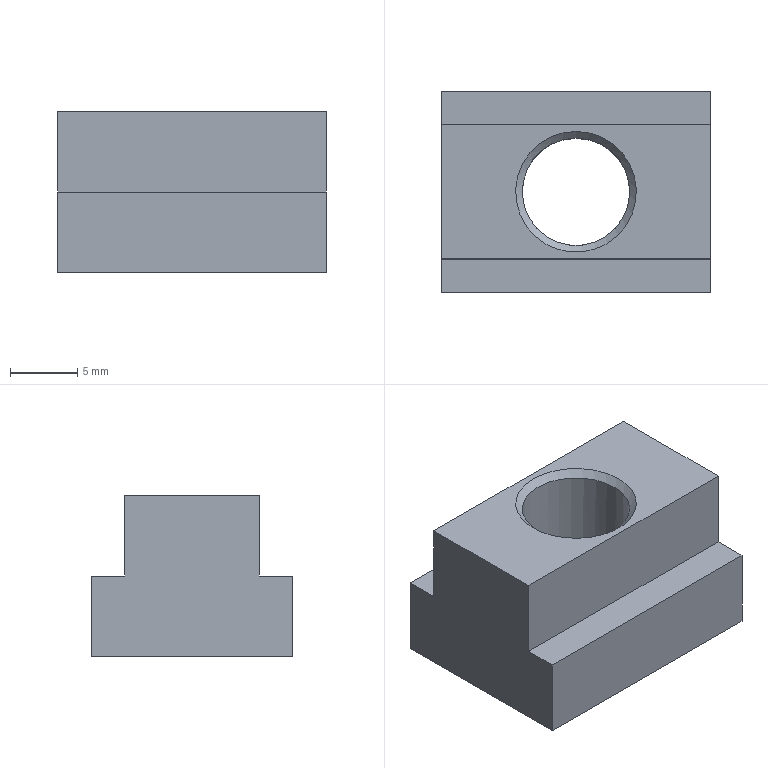Component | NX | FIXED_BLOCK | 1 solid | 13 faces | box 20 x 15 x 12 mm | volume 2390 mm3 | plane 10 | cone 2 | cylinder 1 | commonest cylinder face diameters 8 x1
STEP:
#1=CARTESIAN_POINT('',(0.,0.,0.));
#2=DIRECTION('',(0.,0.,1.));
#3=DIRECTION('',(1.,0.,0.));
#4=AXIS2_PLACEMENT_3D('',#1,#2,#3);
#5=CARTESIAN_POINT('',(-305.,-127.5,4.5));
#6=VERTEX_POINT('',#5);
#7=CARTESIAN_POINT('',(-305.,-127.5,-1.5));
#8=VERTEX_POINT('',#7);
#9=CARTESIAN_POINT('',(-305.,-127.5,4.5));
#10=DIRECTION('',(0.,0.,-1.));
#11=VECTOR('',#10,1.);
#12=LINE('',#9,#11);
#13=CARTESIAN_POINT('',(-285.,-127.5,4.5));
#14=DIRECTION('',(0.,1.,0.));
#15=DIRECTION('',(0.,0.,1.));
#16=AXIS2_PLACEMENT_3D('',#13,#14,#15);
#17=PLANE('',#16);
#18=CARTESIAN_POINT('',(0.,-20.));
#19=DIRECTION('',(-1.,0.));
#20=VECTOR('',#19,1.);
#21=LINE('',#18,#20);
#22=(GEOMETRIC_REPRESENTATION_CONTEXT(2)PARAMETRIC_REPRESENTATION_CONTEXT()REPRESENTATION_CONTEXT('',''));
#23=DEFINITIONAL_REPRESENTATION('',(#21),#22);
#24=PCURVE('',#17,#23);
#25=CARTESIAN_POINT('',(-305.,-120.,10.5));
#26=DIRECTION('',(1.,0.,0.));
#27=DIRECTION('',(0.,0.,-1.));
#28=AXIS2_PLACEMENT_3D('',#25,#26,#27);
#29=PLANE('',#28);
#30=CARTESIAN_POINT('',(6.,-7.5));
#31=DIRECTION('',(1.,0.));
#32=VECTOR('',#31,1.);
#33=LINE('',#30,#32);
#34=(GEOMETRIC_REPRESENTATION_CONTEXT(2)PARAMETRIC_REPRESENTATION_CONTEXT()REPRESENTATION_CONTEXT('',''));
#35=DEFINITIONAL_REPRESENTATION('',(#33),#34);
#36=PCURVE('',#29,#35);
#37=SURFACE_CURVE('',#12,(#24,#36),.PCURVE_S1.);
#38=EDGE_CURVE('',#6,#8,#37,.T.);
#39=ORIENTED_EDGE('',*,*,#38,.T.);
#40=CARTESIAN_POINT('',(-285.,-127.5,-1.5));
#41=VERTEX_POINT('',#40);
#42=CARTESIAN_POINT('',(-285.,-127.5,-1.5));
#43=DIRECTION('',(-1.,0.,0.));
#44=VECTOR('',#43,1.);
#45=LINE('',#42,#44);
#46=CARTESIAN_POINT('',(-6.,0.));
#47=DIRECTION('',(0.,-1.));
#48=VECTOR('',#47,1.);
#49=LINE('',#46,#48);
#50=(GEOMETRIC_REPRESENTATION_CONTEXT(2)PARAMETRIC_REPRESENTATION_CONTEXT()REPRESENTATION_CONTEXT('',''));
#51=DEFINITIONAL_REPRESENTATION('',(#49),#50);
#52=PCURVE('',#17,#51);
#53=CARTESIAN_POINT('',(-285.,-120.,-1.5));
#54=DIRECTION('',(0.,0.,1.));
#55=DIRECTION('',(1.,0.,0.));
#56=AXIS2_PLACEMENT_3D('',#53,#54,#55);
#57=PLANE('',#56);
#58=CARTESIAN_POINT('',(0.,-7.5));
#59=DIRECTION('',(-1.,0.));
#60=VECTOR('',#59,1.);
#61=LINE('',#58,#60);
#62=(GEOMETRIC_REPRESENTATION_CONTEXT(2)PARAMETRIC_REPRESENTATION_CONTEXT()REPRESENTATION_CONTEXT('',''));
#63=DEFINITIONAL_REPRESENTATION('',(#61),#62);
#64=PCURVE('',#57,#63);
#65=SURFACE_CURVE('',#45,(#52,#64),.PCURVE_S1.);
#66=EDGE_CURVE('',#41,#8,#65,.T.);
#67=ORIENTED_EDGE('',*,*,#66,.F.);
#68=CARTESIAN_POINT('',(-285.,-127.5,4.5));
#69=VERTEX_POINT('',#68);
#70=CARTESIAN_POINT('',(-285.,-127.5,4.5));
#71=DIRECTION('',(0.,0.,-1.));
#72=VECTOR('',#71,1.);
#73=LINE('',#70,#72);
#74=CARTESIAN_POINT('',(0.,0.));
#75=DIRECTION('',(-1.,0.));
#76=VECTOR('',#75,1.);
#77=LINE('',#74,#76);
#78=(GEOMETRIC_REPRESENTATION_CONTEXT(2)PARAMETRIC_REPRESENTATION_CONTEXT()REPRESENTATION_CONTEXT('',''));
#79=DEFINITIONAL_REPRESENTATION('',(#77),#78);
#80=PCURVE('',#17,#79);
#81=CARTESIAN_POINT('',(-285.,-120.,10.5));
#82=DIRECTION('',(1.,0.,0.));
#83=DIRECTION('',(0.,0.,-1.));
#84=AXIS2_PLACEMENT_3D('',#81,#82,#83);
#85=PLANE('',#84);
#86=CARTESIAN_POINT('',(6.,-7.5));
#87=DIRECTION('',(1.,0.));
#88=VECTOR('',#87,1.);
#89=LINE('',#86,#88);
#90=(GEOMETRIC_REPRESENTATION_CONTEXT(2)PARAMETRIC_REPRESENTATION_CONTEXT()REPRESENTATION_CONTEXT('',''));
#91=DEFINITIONAL_REPRESENTATION('',(#89),#90);
#92=PCURVE('',#85,#91);
#93=SURFACE_CURVE('',#73,(#80,#92),.PCURVE_S1.);
#94=EDGE_CURVE('',#69,#41,#93,.T.);
#95=ORIENTED_EDGE('',*,*,#94,.F.);
#96=CARTESIAN_POINT('',(-285.,-127.5,4.5));
#97=DIRECTION('',(-1.,0.,0.));
#98=VECTOR('',#97,1.);
#99=LINE('',#96,#98);
#100=CARTESIAN_POINT('',(0.,0.));
#101=DIRECTION('',(0.,-1.));
#102=VECTOR('',#101,1.);
#103=LINE('',#100,#102);
#104=(GEOMETRIC_REPRESENTATION_CONTEXT(2)PARAMETRIC_REPRESENTATION_CONTEXT()REPRESENTATION_CONTEXT('',''));
#105=DEFINITIONAL_REPRESENTATION('',(#103),#104);
#106=PCURVE('',#17,#105);
#107=CARTESIAN_POINT('',(-285.,-125.,4.5));
#108=DIRECTION('',(0.,0.,-1.));
#109=DIRECTION('',(0.,1.,0.));
#110=AXIS2_PLACEMENT_3D('',#107,#108,#109);
#111=PLANE('',#110);
#112=CARTESIAN_POINT('',(-2.5,0.));
#113=DIRECTION('',(0.,-1.));
#114=VECTOR('',#113,1.);
#115=LINE('',#112,#114);
#116=(GEOMETRIC_REPRESENTATION_CONTEXT(2)PARAMETRIC_REPRESENTATION_CONTEXT()REPRESENTATION_CONTEXT('',''));
#117=DEFINITIONAL_REPRESENTATION('',(#115),#116);
#118=PCURVE('',#111,#117);
#119=SURFACE_CURVE('',#99,(#106,#118),.PCURVE_S1.);
#120=EDGE_CURVE('',#69,#6,#119,.T.);
#121=ORIENTED_EDGE('',*,*,#120,.T.);
#122=EDGE_LOOP('',(#39,#67,#95,#121));
#123=FACE_BOUND('',#122,.T.);
#124=ADVANCED_FACE('',(#123),#17,.F.);
#125=CARTESIAN_POINT('',(-290.5,-120.,-1.5));
#126=VERTEX_POINT('',#125);
#127=CARTESIAN_POINT('',(-295.,-115.5,-1.5));
#128=VERTEX_POINT('',#127);
#129=CARTESIAN_POINT('',(-295.,-120.,-1.5));
#130=DIRECTION('',(0.,0.,1.));
#131=DIRECTION('',(1.,0.,0.));
#132=AXIS2_PLACEMENT_3D('',#129,#130,#131);
#133=CIRCLE('',#132,4.5);
#134=CARTESIAN_POINT('',(-10.,0.));
#135=DIRECTION('',(1.,0.));
#136=AXIS2_PLACEMENT_2D('',#134,#135);
#137=CIRCLE('',#136,4.5);
#138=(GEOMETRIC_REPRESENTATION_CONTEXT(2)PARAMETRIC_REPRESENTATION_CONTEXT()REPRESENTATION_CONTEXT('',''));
#139=DEFINITIONAL_REPRESENTATION('',(#137),#138);
#140=PCURVE('',#57,#139);
#141=CARTESIAN_POINT('',(-295.,-120.,-1.5));
#142=DIRECTION('',(0.,0.,-1.));
#143=DIRECTION('',(0.,1.,0.));
#144=AXIS2_PLACEMENT_3D('',#141,#142,#143);
#145=CONICAL_SURFACE('',#144,4.5,0.7854);
#146=CARTESIAN_POINT('',(1.571,0.));
#147=DIRECTION('',(-1.,0.));
#148=VECTOR('',#147,1.);
#149=LINE('',#146,#148);
#150=(GEOMETRIC_REPRESENTATION_CONTEXT(2)PARAMETRIC_REPRESENTATION_CONTEXT()REPRESENTATION_CONTEXT('',''));
#151=DEFINITIONAL_REPRESENTATION('',(#149),#150);
#152=PCURVE('',#145,#151);
#153=SURFACE_CURVE('',#133,(#140,#152),.PCURVE_S1.);
#154=EDGE_CURVE('',#126,#128,#153,.T.);
#155=ORIENTED_EDGE('',*,*,#154,.T.);
#156=CARTESIAN_POINT('',(-295.,-120.,-1.5));
#157=DIRECTION('',(0.,0.,1.));
#158=DIRECTION('',(1.,0.,0.));
#159=AXIS2_PLACEMENT_3D('',#156,#157,#158);
#160=CIRCLE('',#159,4.5);
#161=CARTESIAN_POINT('',(-10.,0.));
#162=DIRECTION('',(1.,0.));
#163=AXIS2_PLACEMENT_2D('',#161,#162);
#164=CIRCLE('',#163,4.5);
#165=(GEOMETRIC_REPRESENTATION_CONTEXT(2)PARAMETRIC_REPRESENTATION_CONTEXT()REPRESENTATION_CONTEXT('',''));
#166=DEFINITIONAL_REPRESENTATION('',(#164),#165);
#167=PCURVE('',#57,#166);
#168=CARTESIAN_POINT('',(7.854,0.));
#169=DIRECTION('',(-1.,0.));
#170=VECTOR('',#169,1.);
#171=LINE('',#168,#170);
#172=(GEOMETRIC_REPRESENTATION_CONTEXT(2)PARAMETRIC_REPRESENTATION_CONTEXT()REPRESENTATION_CONTEXT('',''));
#173=DEFINITIONAL_REPRESENTATION('',(#171),#172);
#174=PCURVE('',#145,#173);
#175=SURFACE_CURVE('',#160,(#167,#174),.PCURVE_S1.);
#176=EDGE_CURVE('',#128,#126,#175,.T.);
#177=ORIENTED_EDGE('',*,*,#176,.T.);
#178=EDGE_LOOP('',(#155,#177));
#179=FACE_BOUND('',#178,.T.);
#180=CARTESIAN_POINT('',(-305.,-112.5,-1.5));
#181=VERTEX_POINT('',#180);
#182=CARTESIAN_POINT('',(-305.,-120.,-1.5));
#183=DIRECTION('',(0.,1.,0.));
#184=VECTOR('',#183,1.);
#185=LINE('',#182,#184);
#186=CARTESIAN_POINT('',(-20.,0.));
#187=DIRECTION('',(0.,1.));
#188=VECTOR('',#187,1.);
#189=LINE('',#186,#188);
#190=(GEOMETRIC_REPRESENTATION_CONTEXT(2)PARAMETRIC_REPRESENTATION_CONTEXT()REPRESENTATION_CONTEXT('',''));
#191=DEFINITIONAL_REPRESENTATION('',(#189),#190);
#192=PCURVE('',#57,#191);
#193=CARTESIAN_POINT('',(12.,0.));
#194=DIRECTION('',(0.,1.));
#195=VECTOR('',#194,1.);
#196=LINE('',#193,#195);
#197=(GEOMETRIC_REPRESENTATION_CONTEXT(2)PARAMETRIC_REPRESENTATION_CONTEXT()REPRESENTATION_CONTEXT('',''));
#198=DEFINITIONAL_REPRESENTATION('',(#196),#197);
#199=PCURVE('',#29,#198);
#200=SURFACE_CURVE('',#185,(#192,#199),.PCURVE_S1.);
#201=EDGE_CURVE('',#8,#181,#200,.T.);
#202=ORIENTED_EDGE('',*,*,#201,.T.);
#203=CARTESIAN_POINT('',(-285.,-112.5,-1.5));
#204=VERTEX_POINT('',#203);
#205=CARTESIAN_POINT('',(-285.,-112.5,-1.5));
#206=DIRECTION('',(-1.,0.,0.));
#207=VECTOR('',#206,1.);
#208=LINE('',#205,#207);
#209=CARTESIAN_POINT('',(0.,7.5));
#210=DIRECTION('',(-1.,0.));
#211=VECTOR('',#210,1.);
#212=LINE('',#209,#211);
#213=(GEOMETRIC_REPRESENTATION_CONTEXT(2)PARAMETRIC_REPRESENTATION_CONTEXT()REPRESENTATION_CONTEXT('',''));
#214=DEFINITIONAL_REPRESENTATION('',(#212),#213);
#215=PCURVE('',#57,#214);
#216=CARTESIAN_POINT('',(-285.,-112.5,-1.5));
#217=DIRECTION('',(0.,-1.,0.));
#218=DIRECTION('',(0.,0.,-1.));
#219=AXIS2_PLACEMENT_3D('',#216,#217,#218);
#220=PLANE('',#219);
#221=CARTESIAN_POINT('',(0.,0.));
#222=DIRECTION('',(0.,-1.));
#223=VECTOR('',#222,1.);
#224=LINE('',#221,#223);
#225=(GEOMETRIC_REPRESENTATION_CONTEXT(2)PARAMETRIC_REPRESENTATION_CONTEXT()REPRESENTATION_CONTEXT('',''));
#226=DEFINITIONAL_REPRESENTATION('',(#224),#225);
#227=PCURVE('',#220,#226);
#228=SURFACE_CURVE('',#208,(#215,#227),.PCURVE_S1.);
#229=EDGE_CURVE('',#204,#181,#228,.T.);
#230=ORIENTED_EDGE('',*,*,#229,.F.);
#231=CARTESIAN_POINT('',(-285.,-127.5,-1.5));
#232=DIRECTION('',(0.,1.,0.));
#233=VECTOR('',#232,1.);
#234=LINE('',#231,#233);
#235=CARTESIAN_POINT('',(0.,-7.5));
#236=DIRECTION('',(0.,1.));
#237=VECTOR('',#236,1.);
#238=LINE('',#235,#237);
#239=(GEOMETRIC_REPRESENTATION_CONTEXT(2)PARAMETRIC_REPRESENTATION_CONTEXT()REPRESENTATION_CONTEXT('',''));
#240=DEFINITIONAL_REPRESENTATION('',(#238),#239);
#241=PCURVE('',#57,#240);
#242=CARTESIAN_POINT('',(12.,-7.5));
#243=DIRECTION('',(0.,1.));
#244=VECTOR('',#243,1.);
#245=LINE('',#242,#244);
#246=(GEOMETRIC_REPRESENTATION_CONTEXT(2)PARAMETRIC_REPRESENTATION_CONTEXT()REPRESENTATION_CONTEXT('',''));
#247=DEFINITIONAL_REPRESENTATION('',(#245),#246);
#248=PCURVE('',#85,#247);
#249=SURFACE_CURVE('',#234,(#241,#248),.PCURVE_S1.);
#250=EDGE_CURVE('',#41,#204,#249,.T.);
#251=ORIENTED_EDGE('',*,*,#250,.F.);
#252=ORIENTED_EDGE('',*,*,#66,.T.);
#253=EDGE_LOOP('',(#202,#230,#251,#252));
#254=FACE_BOUND('',#253,.T.);
#255=ADVANCED_FACE('',(#179,#254),#57,.F.);
#256=CARTESIAN_POINT('',(-305.,-112.5,4.5));
#257=VERTEX_POINT('',#256);
#258=CARTESIAN_POINT('',(-305.,-112.5,-1.5));
#259=DIRECTION('',(0.,0.,1.));
#260=VECTOR('',#259,1.);
#261=LINE('',#258,#260);
#262=CARTESIAN_POINT('',(0.,-20.));
#263=DIRECTION('',(-1.,0.));
#264=VECTOR('',#263,1.);
#265=LINE('',#262,#264);
#266=(GEOMETRIC_REPRESENTATION_CONTEXT(2)PARAMETRIC_REPRESENTATION_CONTEXT()REPRESENTATION_CONTEXT('',''));
#267=DEFINITIONAL_REPRESENTATION('',(#265),#266);
#268=PCURVE('',#220,#267);
#269=CARTESIAN_POINT('',(12.,7.5));
#270=DIRECTION('',(-1.,0.));
#271=VECTOR('',#270,1.);
#272=LINE('',#269,#271);
#273=(GEOMETRIC_REPRESENTATION_CONTEXT(2)PARAMETRIC_REPRESENTATION_CONTEXT()REPRESENTATION_CONTEXT('',''));
#274=DEFINITIONAL_REPRESENTATION('',(#272),#273);
#275=PCURVE('',#29,#274);
#276=SURFACE_CURVE('',#261,(#268,#275),.PCURVE_S1.);
#277=EDGE_CURVE('',#181,#257,#276,.T.);
#278=ORIENTED_EDGE('',*,*,#277,.T.);
#279=CARTESIAN_POINT('',(-285.,-112.5,4.5));
#280=VERTEX_POINT('',#279);
#281=CARTESIAN_POINT('',(-285.,-112.5,4.5));
#282=DIRECTION('',(-1.,0.,0.));
#283=VECTOR('',#282,1.);
#284=LINE('',#281,#283);
#285=CARTESIAN_POINT('',(-6.,0.));
#286=DIRECTION('',(0.,-1.));
#287=VECTOR('',#286,1.);
#288=LINE('',#285,#287);
#289=(GEOMETRIC_REPRESENTATION_CONTEXT(2)PARAMETRIC_REPRESENTATION_CONTEXT()REPRESENTATION_CONTEXT('',''));
#290=DEFINITIONAL_REPRESENTATION('',(#288),#289);
#291=PCURVE('',#220,#290);
#292=CARTESIAN_POINT('',(-285.,-112.5,4.5));
#293=DIRECTION('',(0.,-0.,-1.));
#294=DIRECTION('',(0.,1.,-0.));
#295=AXIS2_PLACEMENT_3D('',#292,#293,#294);
#296=PLANE('',#295);
#297=CARTESIAN_POINT('',(0.,0.));
#298=DIRECTION('',(0.,-1.));
#299=VECTOR('',#298,1.);
#300=LINE('',#297,#299);
#301=(GEOMETRIC_REPRESENTATION_CONTEXT(2)PARAMETRIC_REPRESENTATION_CONTEXT()REPRESENTATION_CONTEXT('',''));
#302=DEFINITIONAL_REPRESENTATION('',(#300),#301);
#303=PCURVE('',#296,#302);
#304=SURFACE_CURVE('',#284,(#291,#303),.PCURVE_S1.);
#305=EDGE_CURVE('',#280,#257,#304,.T.);
#306=ORIENTED_EDGE('',*,*,#305,.F.);
#307=CARTESIAN_POINT('',(-285.,-112.5,-1.5));
#308=DIRECTION('',(0.,0.,1.));
#309=VECTOR('',#308,1.);
#310=LINE('',#307,#309);
#311=CARTESIAN_POINT('',(0.,0.));
#312=DIRECTION('',(-1.,0.));
#313=VECTOR('',#312,1.);
#314=LINE('',#311,#313);
#315=(GEOMETRIC_REPRESENTATION_CONTEXT(2)PARAMETRIC_REPRESENTATION_CONTEXT()REPRESENTATION_CONTEXT('',''));
#316=DEFINITIONAL_REPRESENTATION('',(#314),#315);
#317=PCURVE('',#220,#316);
#318=CARTESIAN_POINT('',(12.,7.5));
#319=DIRECTION('',(-1.,0.));
#320=VECTOR('',#319,1.);
#321=LINE('',#318,#320);
#322=(GEOMETRIC_REPRESENTATION_CONTEXT(2)PARAMETRIC_REPRESENTATION_CONTEXT()REPRESENTATION_CONTEXT('',''));
#323=DEFINITIONAL_REPRESENTATION('',(#321),#322);
#324=PCURVE('',#85,#323);
#325=SURFACE_CURVE('',#310,(#317,#324),.PCURVE_S1.);
#326=EDGE_CURVE('',#204,#280,#325,.T.);
#327=ORIENTED_EDGE('',*,*,#326,.F.);
#328=ORIENTED_EDGE('',*,*,#229,.T.);
#329=EDGE_LOOP('',(#278,#306,#327,#328));
#330=FACE_BOUND('',#329,.T.);
#331=ADVANCED_FACE('',(#330),#220,.F.);
#332=CARTESIAN_POINT('',(-305.,-115.,4.5));
#333=VERTEX_POINT('',#332);
#334=CARTESIAN_POINT('',(-305.,-112.5,4.5));
#335=DIRECTION('',(0.,-1.,0.));
#336=VECTOR('',#335,1.);
#337=LINE('',#334,#336);
#338=CARTESIAN_POINT('',(0.,-20.));
#339=DIRECTION('',(-1.,0.));
#340=VECTOR('',#339,1.);
#341=LINE('',#338,#340);
#342=(GEOMETRIC_REPRESENTATION_CONTEXT(2)PARAMETRIC_REPRESENTATION_CONTEXT()REPRESENTATION_CONTEXT('',''));
#343=DEFINITIONAL_REPRESENTATION('',(#341),#342);
#344=PCURVE('',#296,#343);
#345=CARTESIAN_POINT('',(6.,7.5));
#346=DIRECTION('',(-0.,-1.));
#347=VECTOR('',#346,1.);
#348=LINE('',#345,#347);
#349=(GEOMETRIC_REPRESENTATION_CONTEXT(2)PARAMETRIC_REPRESENTATION_CONTEXT()REPRESENTATION_CONTEXT('',''));
#350=DEFINITIONAL_REPRESENTATION('',(#348),#349);
#351=PCURVE('',#29,#350);
#352=SURFACE_CURVE('',#337,(#344,#351),.PCURVE_S1.);
#353=EDGE_CURVE('',#257,#333,#352,.T.);
#354=ORIENTED_EDGE('',*,*,#353,.T.);
#355=CARTESIAN_POINT('',(-285.,-115.,4.5));
#356=VERTEX_POINT('',#355);
#357=CARTESIAN_POINT('',(-285.,-115.,4.5));
#358=DIRECTION('',(-1.,0.,0.));
#359=VECTOR('',#358,1.);
#360=LINE('',#357,#359);
#361=CARTESIAN_POINT('',(-2.5,0.));
#362=DIRECTION('',(0.,-1.));
#363=VECTOR('',#362,1.);
#364=LINE('',#361,#363);
#365=(GEOMETRIC_REPRESENTATION_CONTEXT(2)PARAMETRIC_REPRESENTATION_CONTEXT()REPRESENTATION_CONTEXT('',''));
#366=DEFINITIONAL_REPRESENTATION('',(#364),#365);
#367=PCURVE('',#296,#366);
#368=CARTESIAN_POINT('',(-285.,-115.,4.5));
#369=DIRECTION('',(0.,-1.,0.));
#370=DIRECTION('',(0.,0.,-1.));
#371=AXIS2_PLACEMENT_3D('',#368,#369,#370);
#372=PLANE('',#371);
#373=CARTESIAN_POINT('',(0.,0.));
#374=DIRECTION('',(0.,-1.));
#375=VECTOR('',#374,1.);
#376=LINE('',#373,#375);
#377=(GEOMETRIC_REPRESENTATION_CONTEXT(2)PARAMETRIC_REPRESENTATION_CONTEXT()REPRESENTATION_CONTEXT('',''));
#378=DEFINITIONAL_REPRESENTATION('',(#376),#377);
#379=PCURVE('',#372,#378);
#380=SURFACE_CURVE('',#360,(#367,#379),.PCURVE_S1.);
#381=EDGE_CURVE('',#356,#333,#380,.T.);
#382=ORIENTED_EDGE('',*,*,#381,.F.);
#383=CARTESIAN_POINT('',(-285.,-112.5,4.5));
#384=DIRECTION('',(0.,-1.,0.));
#385=VECTOR('',#384,1.);
#386=LINE('',#383,#385);
#387=CARTESIAN_POINT('',(0.,0.));
#388=DIRECTION('',(-1.,0.));
#389=VECTOR('',#388,1.);
#390=LINE('',#387,#389);
#391=(GEOMETRIC_REPRESENTATION_CONTEXT(2)PARAMETRIC_REPRESENTATION_CONTEXT()REPRESENTATION_CONTEXT('',''));
#392=DEFINITIONAL_REPRESENTATION('',(#390),#391);
#393=PCURVE('',#296,#392);
#394=CARTESIAN_POINT('',(6.,7.5));
#395=DIRECTION('',(-0.,-1.));
#396=VECTOR('',#395,1.);
#397=LINE('',#394,#396);
#398=(GEOMETRIC_REPRESENTATION_CONTEXT(2)PARAMETRIC_REPRESENTATION_CONTEXT()REPRESENTATION_CONTEXT('',''));
#399=DEFINITIONAL_REPRESENTATION('',(#397),#398);
#400=PCURVE('',#85,#399);
#401=SURFACE_CURVE('',#386,(#393,#400),.PCURVE_S1.);
#402=EDGE_CURVE('',#280,#356,#401,.T.);
#403=ORIENTED_EDGE('',*,*,#402,.F.);
#404=ORIENTED_EDGE('',*,*,#305,.T.);
#405=EDGE_LOOP('',(#354,#382,#403,#404));
#406=FACE_BOUND('',#405,.T.);
#407=ADVANCED_FACE('',(#406),#296,.F.);
#408=CARTESIAN_POINT('',(-305.,-115.,10.5));
#409=VERTEX_POINT('',#408);
#410=CARTESIAN_POINT('',(-305.,-115.,4.5));
#411=DIRECTION('',(0.,0.,1.));
#412=VECTOR('',#411,1.);
#413=LINE('',#410,#412);
#414=CARTESIAN_POINT('',(0.,-20.));
#415=DIRECTION('',(-1.,0.));
#416=VECTOR('',#415,1.);
#417=LINE('',#414,#416);
#418=(GEOMETRIC_REPRESENTATION_CONTEXT(2)PARAMETRIC_REPRESENTATION_CONTEXT()REPRESENTATION_CONTEXT('',''));
#419=DEFINITIONAL_REPRESENTATION('',(#417),#418);
#420=PCURVE('',#372,#419);
#421=CARTESIAN_POINT('',(6.,5.));
#422=DIRECTION('',(-1.,0.));
#423=VECTOR('',#422,1.);
#424=LINE('',#421,#423);
#425=(GEOMETRIC_REPRESENTATION_CONTEXT(2)PARAMETRIC_REPRESENTATION_CONTEXT()REPRESENTATION_CONTEXT('',''));
#426=DEFINITIONAL_REPRESENTATION('',(#424),#425);
#427=PCURVE('',#29,#426);
#428=SURFACE_CURVE('',#413,(#420,#427),.PCURVE_S1.);
#429=EDGE_CURVE('',#333,#409,#428,.T.);
#430=ORIENTED_EDGE('',*,*,#429,.T.);
#431=CARTESIAN_POINT('',(-285.,-115.,10.5));
#432=VERTEX_POINT('',#431);
#433=CARTESIAN_POINT('',(-285.,-115.,10.5));
#434=DIRECTION('',(-1.,0.,0.));
#435=VECTOR('',#434,1.);
#436=LINE('',#433,#435);
#437=CARTESIAN_POINT('',(-6.,0.));
#438=DIRECTION('',(0.,-1.));
#439=VECTOR('',#438,1.);
#440=LINE('',#437,#439);
#441=(GEOMETRIC_REPRESENTATION_CONTEXT(2)PARAMETRIC_REPRESENTATION_CONTEXT()REPRESENTATION_CONTEXT('',''));
#442=DEFINITIONAL_REPRESENTATION('',(#440),#441);
#443=PCURVE('',#372,#442);
#444=CARTESIAN_POINT('',(-285.,-120.,10.5));
#445=DIRECTION('',(0.,0.,-1.));
#446=DIRECTION('',(0.,1.,0.));
#447=AXIS2_PLACEMENT_3D('',#444,#445,#446);
#448=PLANE('',#447);
#449=CARTESIAN_POINT('',(5.,0.));
#450=DIRECTION('',(0.,-1.));
#451=VECTOR('',#450,1.);
#452=LINE('',#449,#451);
#453=(GEOMETRIC_REPRESENTATION_CONTEXT(2)PARAMETRIC_REPRESENTATION_CONTEXT()REPRESENTATION_CONTEXT('',''));
#454=DEFINITIONAL_REPRESENTATION('',(#452),#453);
#455=PCURVE('',#448,#454);
#456=SURFACE_CURVE('',#436,(#443,#455),.PCURVE_S1.);
#457=EDGE_CURVE('',#432,#409,#456,.T.);
#458=ORIENTED_EDGE('',*,*,#457,.F.);
#459=CARTESIAN_POINT('',(-285.,-115.,4.5));
#460=DIRECTION('',(0.,0.,1.));
#461=VECTOR('',#460,1.);
#462=LINE('',#459,#461);
#463=CARTESIAN_POINT('',(0.,0.));
#464=DIRECTION('',(-1.,0.));
#465=VECTOR('',#464,1.);
#466=LINE('',#463,#465);
#467=(GEOMETRIC_REPRESENTATION_CONTEXT(2)PARAMETRIC_REPRESENTATION_CONTEXT()REPRESENTATION_CONTEXT('',''));
#468=DEFINITIONAL_REPRESENTATION('',(#466),#467);
#469=PCURVE('',#372,#468);
#470=CARTESIAN_POINT('',(6.,5.));
#471=DIRECTION('',(-1.,0.));
#472=VECTOR('',#471,1.);
#473=LINE('',#470,#472);
#474=(GEOMETRIC_REPRESENTATION_CONTEXT(2)PARAMETRIC_REPRESENTATION_CONTEXT()REPRESENTATION_CONTEXT('',''));
#475=DEFINITIONAL_REPRESENTATION('',(#473),#474);
#476=PCURVE('',#85,#475);
#477=SURFACE_CURVE('',#462,(#469,#476),.PCURVE_S1.);
#478=EDGE_CURVE('',#356,#432,#477,.T.);
#479=ORIENTED_EDGE('',*,*,#478,.F.);
#480=ORIENTED_EDGE('',*,*,#381,.T.);
#481=EDGE_LOOP('',(#430,#458,#479,#480));
#482=FACE_BOUND('',#481,.T.);
#483=ADVANCED_FACE('',(#482),#372,.F.);
#484=CARTESIAN_POINT('',(-295.,-115.5,10.5));
#485=VERTEX_POINT('',#484);
#486=CARTESIAN_POINT('',(-295.,-120.,10.5));
#487=DIRECTION('',(0.,0.,-1.));
#488=DIRECTION('',(0.,1.,0.));
#489=AXIS2_PLACEMENT_3D('',#486,#487,#488);
#490=CIRCLE('',#489,4.5);
#491=CARTESIAN_POINT('',(0.,-10.));
#492=DIRECTION('',(1.,0.));
#493=AXIS2_PLACEMENT_2D('',#491,#492);
#494=CIRCLE('',#493,4.5);
#495=(GEOMETRIC_REPRESENTATION_CONTEXT(2)PARAMETRIC_REPRESENTATION_CONTEXT()REPRESENTATION_CONTEXT('',''));
#496=DEFINITIONAL_REPRESENTATION('',(#494),#495);
#497=PCURVE('',#448,#496);
#498=CARTESIAN_POINT('',(-295.,-120.,10.5));
#499=DIRECTION('',(0.,-0.,1.));
#500=DIRECTION('',(0.,-1.,-0.));
#501=AXIS2_PLACEMENT_3D('',#498,#499,#500);
#502=CONICAL_SURFACE('',#501,4.5,0.7854);
#503=CARTESIAN_POINT('',(9.425,0.));
#504=DIRECTION('',(-1.,0.));
#505=VECTOR('',#504,1.);
#506=LINE('',#503,#505);
#507=(GEOMETRIC_REPRESENTATION_CONTEXT(2)PARAMETRIC_REPRESENTATION_CONTEXT()REPRESENTATION_CONTEXT('',''));
#508=DEFINITIONAL_REPRESENTATION('',(#506),#507);
#509=PCURVE('',#502,#508);
#510=SURFACE_CURVE('',#490,(#497,#509),.PCURVE_S1.);
#511=EDGE_CURVE('',#485,#485,#510,.T.);
#512=ORIENTED_EDGE('',*,*,#511,.T.);
#513=EDGE_LOOP('',(#512));
#514=FACE_BOUND('',#513,.T.);
#515=CARTESIAN_POINT('',(-305.,-125.,10.5));
#516=VERTEX_POINT('',#515);
#517=CARTESIAN_POINT('',(-305.,-120.,10.5));
#518=DIRECTION('',(0.,-1.,-0.));
#519=VECTOR('',#518,1.);
#520=LINE('',#517,#519);
#521=CARTESIAN_POINT('',(0.,-20.));
#522=DIRECTION('',(-1.,0.));
#523=VECTOR('',#522,1.);
#524=LINE('',#521,#523);
#525=(GEOMETRIC_REPRESENTATION_CONTEXT(2)PARAMETRIC_REPRESENTATION_CONTEXT()REPRESENTATION_CONTEXT('',''));
#526=DEFINITIONAL_REPRESENTATION('',(#524),#525);
#527=PCURVE('',#448,#526);
#528=CARTESIAN_POINT('',(0.,0.));
#529=DIRECTION('',(0.,-1.));
#530=VECTOR('',#529,1.);
#531=LINE('',#528,#530);
#532=(GEOMETRIC_REPRESENTATION_CONTEXT(2)PARAMETRIC_REPRESENTATION_CONTEXT()REPRESENTATION_CONTEXT('',''));
#533=DEFINITIONAL_REPRESENTATION('',(#531),#532);
#534=PCURVE('',#29,#533);
#535=SURFACE_CURVE('',#520,(#527,#534),.PCURVE_S1.);
#536=EDGE_CURVE('',#409,#516,#535,.T.);
#537=ORIENTED_EDGE('',*,*,#536,.T.);
#538=CARTESIAN_POINT('',(-285.,-125.,10.5));
#539=VERTEX_POINT('',#538);
#540=CARTESIAN_POINT('',(-285.,-125.,10.5));
#541=DIRECTION('',(-1.,0.,0.));
#542=VECTOR('',#541,1.);
#543=LINE('',#540,#542);
#544=CARTESIAN_POINT('',(-5.,0.));
#545=DIRECTION('',(0.,-1.));
#546=VECTOR('',#545,1.);
#547=LINE('',#544,#546);
#548=(GEOMETRIC_REPRESENTATION_CONTEXT(2)PARAMETRIC_REPRESENTATION_CONTEXT()REPRESENTATION_CONTEXT('',''));
#549=DEFINITIONAL_REPRESENTATION('',(#547),#548);
#550=PCURVE('',#448,#549);
#551=CARTESIAN_POINT('',(-285.,-125.,10.5));
#552=DIRECTION('',(0.,1.,0.));
#553=DIRECTION('',(0.,0.,1.));
#554=AXIS2_PLACEMENT_3D('',#551,#552,#553);
#555=PLANE('',#554);
#556=CARTESIAN_POINT('',(0.,0.));
#557=DIRECTION('',(0.,-1.));
#558=VECTOR('',#557,1.);
#559=LINE('',#556,#558);
#560=(GEOMETRIC_REPRESENTATION_CONTEXT(2)PARAMETRIC_REPRESENTATION_CONTEXT()REPRESENTATION_CONTEXT('',''));
#561=DEFINITIONAL_REPRESENTATION('',(#559),#560);
#562=PCURVE('',#555,#561);
#563=SURFACE_CURVE('',#543,(#550,#562),.PCURVE_S1.);
#564=EDGE_CURVE('',#539,#516,#563,.T.);
#565=ORIENTED_EDGE('',*,*,#564,.F.);
#566=CARTESIAN_POINT('',(-285.,-115.,10.5));
#567=DIRECTION('',(0.,-1.,0.));
#568=VECTOR('',#567,1.);
#569=LINE('',#566,#568);
#570=CARTESIAN_POINT('',(5.,0.));
#571=DIRECTION('',(-1.,0.));
#572=VECTOR('',#571,1.);
#573=LINE('',#570,#572);
#574=(GEOMETRIC_REPRESENTATION_CONTEXT(2)PARAMETRIC_REPRESENTATION_CONTEXT()REPRESENTATION_CONTEXT('',''));
#575=DEFINITIONAL_REPRESENTATION('',(#573),#574);
#576=PCURVE('',#448,#575);
#577=CARTESIAN_POINT('',(0.,5.));
#578=DIRECTION('',(-0.,-1.));
#579=VECTOR('',#578,1.);
#580=LINE('',#577,#579);
#581=(GEOMETRIC_REPRESENTATION_CONTEXT(2)PARAMETRIC_REPRESENTATION_CONTEXT()REPRESENTATION_CONTEXT('',''));
#582=DEFINITIONAL_REPRESENTATION('',(#580),#581);
#583=PCURVE('',#85,#582);
#584=SURFACE_CURVE('',#569,(#576,#583),.PCURVE_S1.);
#585=EDGE_CURVE('',#432,#539,#584,.T.);
#586=ORIENTED_EDGE('',*,*,#585,.F.);
#587=ORIENTED_EDGE('',*,*,#457,.T.);
#588=EDGE_LOOP('',(#537,#565,#586,#587));
#589=FACE_BOUND('',#588,.T.);
#590=ADVANCED_FACE('',(#514,#589),#448,.F.);
#591=CARTESIAN_POINT('',(-305.,-125.,4.5));
#592=VERTEX_POINT('',#591);
#593=CARTESIAN_POINT('',(-305.,-125.,10.5));
#594=DIRECTION('',(0.,0.,-1.));
#595=VECTOR('',#594,1.);
#596=LINE('',#593,#595);
#597=CARTESIAN_POINT('',(0.,-20.));
#598=DIRECTION('',(-1.,0.));
#599=VECTOR('',#598,1.);
#600=LINE('',#597,#599);
#601=(GEOMETRIC_REPRESENTATION_CONTEXT(2)PARAMETRIC_REPRESENTATION_CONTEXT()REPRESENTATION_CONTEXT('',''));
#602=DEFINITIONAL_REPRESENTATION('',(#600),#601);
#603=PCURVE('',#555,#602);
#604=CARTESIAN_POINT('',(0.,-5.));
#605=DIRECTION('',(1.,0.));
#606=VECTOR('',#605,1.);
#607=LINE('',#604,#606);
#608=(GEOMETRIC_REPRESENTATION_CONTEXT(2)PARAMETRIC_REPRESENTATION_CONTEXT()REPRESENTATION_CONTEXT('',''));
#609=DEFINITIONAL_REPRESENTATION('',(#607),#608);
#610=PCURVE('',#29,#609);
#611=SURFACE_CURVE('',#596,(#603,#610),.PCURVE_S1.);
#612=EDGE_CURVE('',#516,#592,#611,.T.);
#613=ORIENTED_EDGE('',*,*,#612,.T.);
#614=CARTESIAN_POINT('',(-285.,-125.,4.5));
#615=VERTEX_POINT('',#614);
#616=CARTESIAN_POINT('',(-285.,-125.,4.5));
#617=DIRECTION('',(-1.,0.,0.));
#618=VECTOR('',#617,1.);
#619=LINE('',#616,#618);
#620=CARTESIAN_POINT('',(-6.,0.));
#621=DIRECTION('',(0.,-1.));
#622=VECTOR('',#621,1.);
#623=LINE('',#620,#622);
#624=(GEOMETRIC_REPRESENTATION_CONTEXT(2)PARAMETRIC_REPRESENTATION_CONTEXT()REPRESENTATION_CONTEXT('',''));
#625=DEFINITIONAL_REPRESENTATION('',(#623),#624);
#626=PCURVE('',#555,#625);
#627=CARTESIAN_POINT('',(0.,0.));
#628=DIRECTION('',(0.,-1.));
#629=VECTOR('',#628,1.);
#630=LINE('',#627,#629);
#631=(GEOMETRIC_REPRESENTATION_CONTEXT(2)PARAMETRIC_REPRESENTATION_CONTEXT()REPRESENTATION_CONTEXT('',''));
#632=DEFINITIONAL_REPRESENTATION('',(#630),#631);
#633=PCURVE('',#111,#632);
#634=SURFACE_CURVE('',#619,(#626,#633),.PCURVE_S1.);
#635=EDGE_CURVE('',#615,#592,#634,.T.);
#636=ORIENTED_EDGE('',*,*,#635,.F.);
#637=CARTESIAN_POINT('',(-285.,-125.,10.5));
#638=DIRECTION('',(0.,0.,-1.));
#639=VECTOR('',#638,1.);
#640=LINE('',#637,#639);
#641=CARTESIAN_POINT('',(0.,0.));
#642=DIRECTION('',(-1.,0.));
#643=VECTOR('',#642,1.);
#644=LINE('',#641,#643);
#645=(GEOMETRIC_REPRESENTATION_CONTEXT(2)PARAMETRIC_REPRESENTATION_CONTEXT()REPRESENTATION_CONTEXT('',''));
#646=DEFINITIONAL_REPRESENTATION('',(#644),#645);
#647=PCURVE('',#555,#646);
#648=CARTESIAN_POINT('',(0.,-5.));
#649=DIRECTION('',(1.,0.));
#650=VECTOR('',#649,1.);
#651=LINE('',#648,#650);
#652=(GEOMETRIC_REPRESENTATION_CONTEXT(2)PARAMETRIC_REPRESENTATION_CONTEXT()REPRESENTATION_CONTEXT('',''));
#653=DEFINITIONAL_REPRESENTATION('',(#651),#652);
#654=PCURVE('',#85,#653);
#655=SURFACE_CURVE('',#640,(#647,#654),.PCURVE_S1.);
#656=EDGE_CURVE('',#539,#615,#655,.T.);
#657=ORIENTED_EDGE('',*,*,#656,.F.);
#658=ORIENTED_EDGE('',*,*,#564,.T.);
#659=EDGE_LOOP('',(#613,#636,#657,#658));
#660=FACE_BOUND('',#659,.T.);
#661=ADVANCED_FACE('',(#660),#555,.F.);
#662=CARTESIAN_POINT('',(-305.,-125.,4.5));
#663=DIRECTION('',(0.,-1.,-0.));
#664=VECTOR('',#663,1.);
#665=LINE('',#662,#664);
#666=CARTESIAN_POINT('',(0.,-20.));
#667=DIRECTION('',(-1.,0.));
#668=VECTOR('',#667,1.);
#669=LINE('',#666,#668);
#670=(GEOMETRIC_REPRESENTATION_CONTEXT(2)PARAMETRIC_REPRESENTATION_CONTEXT()REPRESENTATION_CONTEXT('',''));
#671=DEFINITIONAL_REPRESENTATION('',(#669),#670);
#672=PCURVE('',#111,#671);
#673=CARTESIAN_POINT('',(6.,-5.));
#674=DIRECTION('',(0.,-1.));
#675=VECTOR('',#674,1.);
#676=LINE('',#673,#675);
#677=(GEOMETRIC_REPRESENTATION_CONTEXT(2)PARAMETRIC_REPRESENTATION_CONTEXT()REPRESENTATION_CONTEXT('',''));
#678=DEFINITIONAL_REPRESENTATION('',(#676),#677);
#679=PCURVE('',#29,#678);
#680=SURFACE_CURVE('',#665,(#672,#679),.PCURVE_S1.);
#681=EDGE_CURVE('',#592,#6,#680,.T.);
#682=ORIENTED_EDGE('',*,*,#681,.T.);
#683=ORIENTED_EDGE('',*,*,#120,.F.);
#684=CARTESIAN_POINT('',(-285.,-125.,4.5));
#685=DIRECTION('',(0.,-1.,-0.));
#686=VECTOR('',#685,1.);
#687=LINE('',#684,#686);
#688=CARTESIAN_POINT('',(0.,0.));
#689=DIRECTION('',(-1.,0.));
#690=VECTOR('',#689,1.);
#691=LINE('',#688,#690);
#692=(GEOMETRIC_REPRESENTATION_CONTEXT(2)PARAMETRIC_REPRESENTATION_CONTEXT()REPRESENTATION_CONTEXT('',''));
#693=DEFINITIONAL_REPRESENTATION('',(#691),#692);
#694=PCURVE('',#111,#693);
#695=CARTESIAN_POINT('',(6.,-5.));
#696=DIRECTION('',(0.,-1.));
#697=VECTOR('',#696,1.);
#698=LINE('',#695,#697);
#699=(GEOMETRIC_REPRESENTATION_CONTEXT(2)PARAMETRIC_REPRESENTATION_CONTEXT()REPRESENTATION_CONTEXT('',''));
#700=DEFINITIONAL_REPRESENTATION('',(#698),#699);
#701=PCURVE('',#85,#700);
#702=SURFACE_CURVE('',#687,(#694,#701),.PCURVE_S1.);
#703=EDGE_CURVE('',#615,#69,#702,.T.);
#704=ORIENTED_EDGE('',*,*,#703,.F.);
#705=ORIENTED_EDGE('',*,*,#635,.T.);
#706=EDGE_LOOP('',(#682,#683,#704,#705));
#707=FACE_BOUND('',#706,.T.);
#708=ADVANCED_FACE('',(#707),#111,.F.);
#709=ORIENTED_EDGE('',*,*,#94,.T.);
#710=ORIENTED_EDGE('',*,*,#250,.T.);
#711=ORIENTED_EDGE('',*,*,#326,.T.);
#712=ORIENTED_EDGE('',*,*,#402,.T.);
#713=ORIENTED_EDGE('',*,*,#478,.T.);
#714=ORIENTED_EDGE('',*,*,#585,.T.);
#715=ORIENTED_EDGE('',*,*,#656,.T.);
#716=ORIENTED_EDGE('',*,*,#703,.T.);
#717=EDGE_LOOP('',(#709,#710,#711,#712,#713,#714,#715,#716));
#718=FACE_BOUND('',#717,.T.);
#719=ADVANCED_FACE('',(#718),#85,.T.);
#720=ORIENTED_EDGE('',*,*,#38,.F.);
#721=ORIENTED_EDGE('',*,*,#681,.F.);
#722=ORIENTED_EDGE('',*,*,#612,.F.);
#723=ORIENTED_EDGE('',*,*,#536,.F.);
#724=ORIENTED_EDGE('',*,*,#429,.F.);
#725=ORIENTED_EDGE('',*,*,#353,.F.);
#726=ORIENTED_EDGE('',*,*,#277,.F.);
#727=ORIENTED_EDGE('',*,*,#201,.F.);
#728=EDGE_LOOP('',(#720,#721,#722,#723,#724,#725,#726,#727));
#729=FACE_BOUND('',#728,.T.);
#730=ADVANCED_FACE('',(#729),#29,.F.);
#731=CARTESIAN_POINT('',(-295.,-116.,-1.));
#732=VERTEX_POINT('',#731);
#733=CARTESIAN_POINT('',(-295.,-124.,-1.));
#734=VERTEX_POINT('',#733);
#735=CARTESIAN_POINT('',(-295.,-120.,-1.));
#736=DIRECTION('',(0.,0.,-1.));
#737=DIRECTION('',(0.,-1.,-0.));
#738=AXIS2_PLACEMENT_3D('',#735,#736,#737);
#739=CIRCLE('',#738,4.);
#740=CARTESIAN_POINT('',(-295.,-120.,10.5));
#741=DIRECTION('',(0.,0.,-1.));
#742=DIRECTION('',(0.,1.,0.));
#743=AXIS2_PLACEMENT_3D('',#740,#741,#742);
#744=CYLINDRICAL_SURFACE('',#743,4.);
#745=CARTESIAN_POINT('',(-3.142,11.5));
#746=DIRECTION('',(1.,0.));
#747=VECTOR('',#746,1.);
#748=LINE('',#745,#747);
#749=(GEOMETRIC_REPRESENTATION_CONTEXT(2)PARAMETRIC_REPRESENTATION_CONTEXT()REPRESENTATION_CONTEXT('',''));
#750=DEFINITIONAL_REPRESENTATION('',(#748),#749);
#751=PCURVE('',#744,#750);
#752=CARTESIAN_POINT('',(-3.142,-0.5));
#753=DIRECTION('',(1.,0.));
#754=VECTOR('',#753,1.);
#755=LINE('',#752,#754);
#756=(GEOMETRIC_REPRESENTATION_CONTEXT(2)PARAMETRIC_REPRESENTATION_CONTEXT()REPRESENTATION_CONTEXT('',''));
#757=DEFINITIONAL_REPRESENTATION('',(#755),#756);
#758=PCURVE('',#145,#757);
#759=SURFACE_CURVE('',#739,(#751,#758),.PCURVE_S1.);
#760=EDGE_CURVE('',#732,#734,#759,.T.);
#761=ORIENTED_EDGE('',*,*,#760,.F.);
#762=CARTESIAN_POINT('',(-295.,-116.,10.));
#763=VERTEX_POINT('',#762);
#764=CARTESIAN_POINT('',(-295.,-116.,10.));
#765=CARTESIAN_POINT('',(-295.,-116.,-1.));
#766=B_SPLINE_CURVE_WITH_KNOTS('',1,(#764,#765),.UNSPECIFIED.,.F.,.F.,(2,2),(0.5,11.5),.PIECEWISE_BEZIER_KNOTS.);
#767=CARTESIAN_POINT('',(0.,0.));
#768=DIRECTION('',(0.,1.));
#769=VECTOR('',#768,1.);
#770=LINE('',#767,#769);
#771=(GEOMETRIC_REPRESENTATION_CONTEXT(2)PARAMETRIC_REPRESENTATION_CONTEXT()REPRESENTATION_CONTEXT('',''));
#772=DEFINITIONAL_REPRESENTATION('',(#770),#771);
#773=PCURVE('',#744,#772);
#774=CARTESIAN_POINT('',(6.283,0.));
#775=DIRECTION('',(0.,1.));
#776=VECTOR('',#775,1.);
#777=LINE('',#774,#776);
#778=(GEOMETRIC_REPRESENTATION_CONTEXT(2)PARAMETRIC_REPRESENTATION_CONTEXT()REPRESENTATION_CONTEXT('',''));
#779=DEFINITIONAL_REPRESENTATION('',(#777),#778);
#780=PCURVE('',#744,#779);
#781=SEAM_CURVE('',#766,(#773,#780),.PCURVE_S1.);
#782=EDGE_CURVE('',#763,#732,#781,.T.);
#783=ORIENTED_EDGE('',*,*,#782,.F.);
#784=CARTESIAN_POINT('',(-295.,-120.,10.));
#785=DIRECTION('',(0.,-0.,1.));
#786=DIRECTION('',(0.,1.,0.));
#787=AXIS2_PLACEMENT_3D('',#784,#785,#786);
#788=CIRCLE('',#787,4.);
#789=CARTESIAN_POINT('',(6.283,0.5));
#790=DIRECTION('',(-1.,0.));
#791=VECTOR('',#790,1.);
#792=LINE('',#789,#791);
#793=(GEOMETRIC_REPRESENTATION_CONTEXT(2)PARAMETRIC_REPRESENTATION_CONTEXT()REPRESENTATION_CONTEXT('',''));
#794=DEFINITIONAL_REPRESENTATION('',(#792),#793);
#795=PCURVE('',#744,#794);
#796=CARTESIAN_POINT('',(3.142,-0.5));
#797=DIRECTION('',(1.,0.));
#798=VECTOR('',#797,1.);
#799=LINE('',#796,#798);
#800=(GEOMETRIC_REPRESENTATION_CONTEXT(2)PARAMETRIC_REPRESENTATION_CONTEXT()REPRESENTATION_CONTEXT('',''));
#801=DEFINITIONAL_REPRESENTATION('',(#799),#800);
#802=PCURVE('',#502,#801);
#803=SURFACE_CURVE('',#788,(#795,#802),.PCURVE_S1.);
#804=EDGE_CURVE('',#763,#763,#803,.T.);
#805=ORIENTED_EDGE('',*,*,#804,.F.);
#806=ORIENTED_EDGE('',*,*,#782,.T.);
#807=CARTESIAN_POINT('',(-295.,-120.,-1.));
#808=DIRECTION('',(0.,0.,-1.));
#809=DIRECTION('',(0.,-1.,-0.));
#810=AXIS2_PLACEMENT_3D('',#807,#808,#809);
#811=CIRCLE('',#810,4.);
#812=CARTESIAN_POINT('',(3.142,11.5));
#813=DIRECTION('',(1.,0.));
#814=VECTOR('',#813,1.);
#815=LINE('',#812,#814);
#816=(GEOMETRIC_REPRESENTATION_CONTEXT(2)PARAMETRIC_REPRESENTATION_CONTEXT()REPRESENTATION_CONTEXT('',''));
#817=DEFINITIONAL_REPRESENTATION('',(#815),#816);
#818=PCURVE('',#744,#817);
#819=CARTESIAN_POINT('',(3.142,-0.5));
#820=DIRECTION('',(1.,0.));
#821=VECTOR('',#820,1.);
#822=LINE('',#819,#821);
#823=(GEOMETRIC_REPRESENTATION_CONTEXT(2)PARAMETRIC_REPRESENTATION_CONTEXT()REPRESENTATION_CONTEXT('',''));
#824=DEFINITIONAL_REPRESENTATION('',(#822),#823);
#825=PCURVE('',#145,#824);
#826=SURFACE_CURVE('',#811,(#818,#825),.PCURVE_S1.);
#827=EDGE_CURVE('',#734,#732,#826,.T.);
#828=ORIENTED_EDGE('',*,*,#827,.F.);
#829=EDGE_LOOP('',(#761,#783,#805,#806,#828));
#830=FACE_BOUND('',#829,.F.);
#831=ADVANCED_FACE('',(#830),#744,.F.);
#832=ORIENTED_EDGE('',*,*,#804,.T.);
#833=CARTESIAN_POINT('',(-295.,-116.,10.));
#834=CARTESIAN_POINT('',(-295.,-115.5,10.5));
#835=B_SPLINE_CURVE_WITH_KNOTS('',1,(#833,#834),.UNSPECIFIED.,.F.,.F.,(2,2),(-0.7071,0.),.PIECEWISE_BEZIER_KNOTS.);
#836=CARTESIAN_POINT('',(9.425,0.));
#837=DIRECTION('',(0.,1.));
#838=VECTOR('',#837,1.);
#839=LINE('',#836,#838);
#840=(GEOMETRIC_REPRESENTATION_CONTEXT(2)PARAMETRIC_REPRESENTATION_CONTEXT()REPRESENTATION_CONTEXT('',''));
#841=DEFINITIONAL_REPRESENTATION('',(#839),#840);
#842=PCURVE('',#502,#841);
#843=CARTESIAN_POINT('',(3.142,0.));
#844=DIRECTION('',(0.,1.));
#845=VECTOR('',#844,1.);
#846=LINE('',#843,#845);
#847=(GEOMETRIC_REPRESENTATION_CONTEXT(2)PARAMETRIC_REPRESENTATION_CONTEXT()REPRESENTATION_CONTEXT('',''));
#848=DEFINITIONAL_REPRESENTATION('',(#846),#847);
#849=PCURVE('',#502,#848);
#850=SEAM_CURVE('',#835,(#842,#849),.PCURVE_S1.);
#851=EDGE_CURVE('',#763,#485,#850,.T.);
#852=ORIENTED_EDGE('',*,*,#851,.T.);
#853=ORIENTED_EDGE('',*,*,#511,.T.);
#854=ORIENTED_EDGE('',*,*,#851,.F.);
#855=EDGE_LOOP('',(#832,#852,#853,#854));
#856=FACE_BOUND('',#855,.F.);
#857=ADVANCED_FACE('',(#856),#502,.F.);
#858=ORIENTED_EDGE('',*,*,#760,.T.);
#859=ORIENTED_EDGE('',*,*,#827,.T.);
#860=CARTESIAN_POINT('',(-295.,-116.,-1.));
#861=CARTESIAN_POINT('',(-295.,-115.5,-1.5));
#862=B_SPLINE_CURVE_WITH_KNOTS('',1,(#860,#861),.UNSPECIFIED.,.F.,.F.,(2,2),(-0.7071,0.),.PIECEWISE_BEZIER_KNOTS.);
#863=CARTESIAN_POINT('',(6.283,0.));
#864=DIRECTION('',(0.,1.));
#865=VECTOR('',#864,1.);
#866=LINE('',#863,#865);
#867=(GEOMETRIC_REPRESENTATION_CONTEXT(2)PARAMETRIC_REPRESENTATION_CONTEXT()REPRESENTATION_CONTEXT('',''));
#868=DEFINITIONAL_REPRESENTATION('',(#866),#867);
#869=PCURVE('',#145,#868);
#870=CARTESIAN_POINT('',(0.,0.));
#871=DIRECTION('',(0.,1.));
#872=VECTOR('',#871,1.);
#873=LINE('',#870,#872);
#874=(GEOMETRIC_REPRESENTATION_CONTEXT(2)PARAMETRIC_REPRESENTATION_CONTEXT()REPRESENTATION_CONTEXT('',''));
#875=DEFINITIONAL_REPRESENTATION('',(#873),#874);
#876=PCURVE('',#145,#875);
#877=SEAM_CURVE('',#862,(#869,#876),.PCURVE_S1.);
#878=EDGE_CURVE('',#732,#128,#877,.T.);
#879=ORIENTED_EDGE('',*,*,#878,.T.);
#880=ORIENTED_EDGE('',*,*,#176,.T.);
#881=ORIENTED_EDGE('',*,*,#154,.T.);
#882=ORIENTED_EDGE('',*,*,#878,.F.);
#883=EDGE_LOOP('',(#858,#859,#879,#880,#881,#882));
#884=FACE_BOUND('',#883,.F.);
#885=ADVANCED_FACE('',(#884),#145,.F.);
#886=CLOSED_SHELL('',(#124,#255,#331,#407,#483,#590,#661,#708,#719,#730,#831,#857,#885));
#887=MANIFOLD_SOLID_BREP('',#886);
#888=(LENGTH_UNIT()NAMED_UNIT(*)SI_UNIT(.MILLI.,.METRE.));
#889=UNCERTAINTY_MEASURE_WITH_UNIT(LENGTH_MEASURE(0.000002),#888,'','');
#890=(NAMED_UNIT(*)PLANE_ANGLE_UNIT()SI_UNIT($,.RADIAN.));
#891=(NAMED_UNIT(*)SI_UNIT($,.STERADIAN.)SOLID_ANGLE_UNIT());
#892=(GEOMETRIC_REPRESENTATION_CONTEXT(3)GLOBAL_UNCERTAINTY_ASSIGNED_CONTEXT((#889))GLOBAL_UNIT_ASSIGNED_CONTEXT((#888,#890,#891))REPRESENTATION_CONTEXT('',''));
#893=ADVANCED_BREP_SHAPE_REPRESENTATION('',(#4,#887),#892);